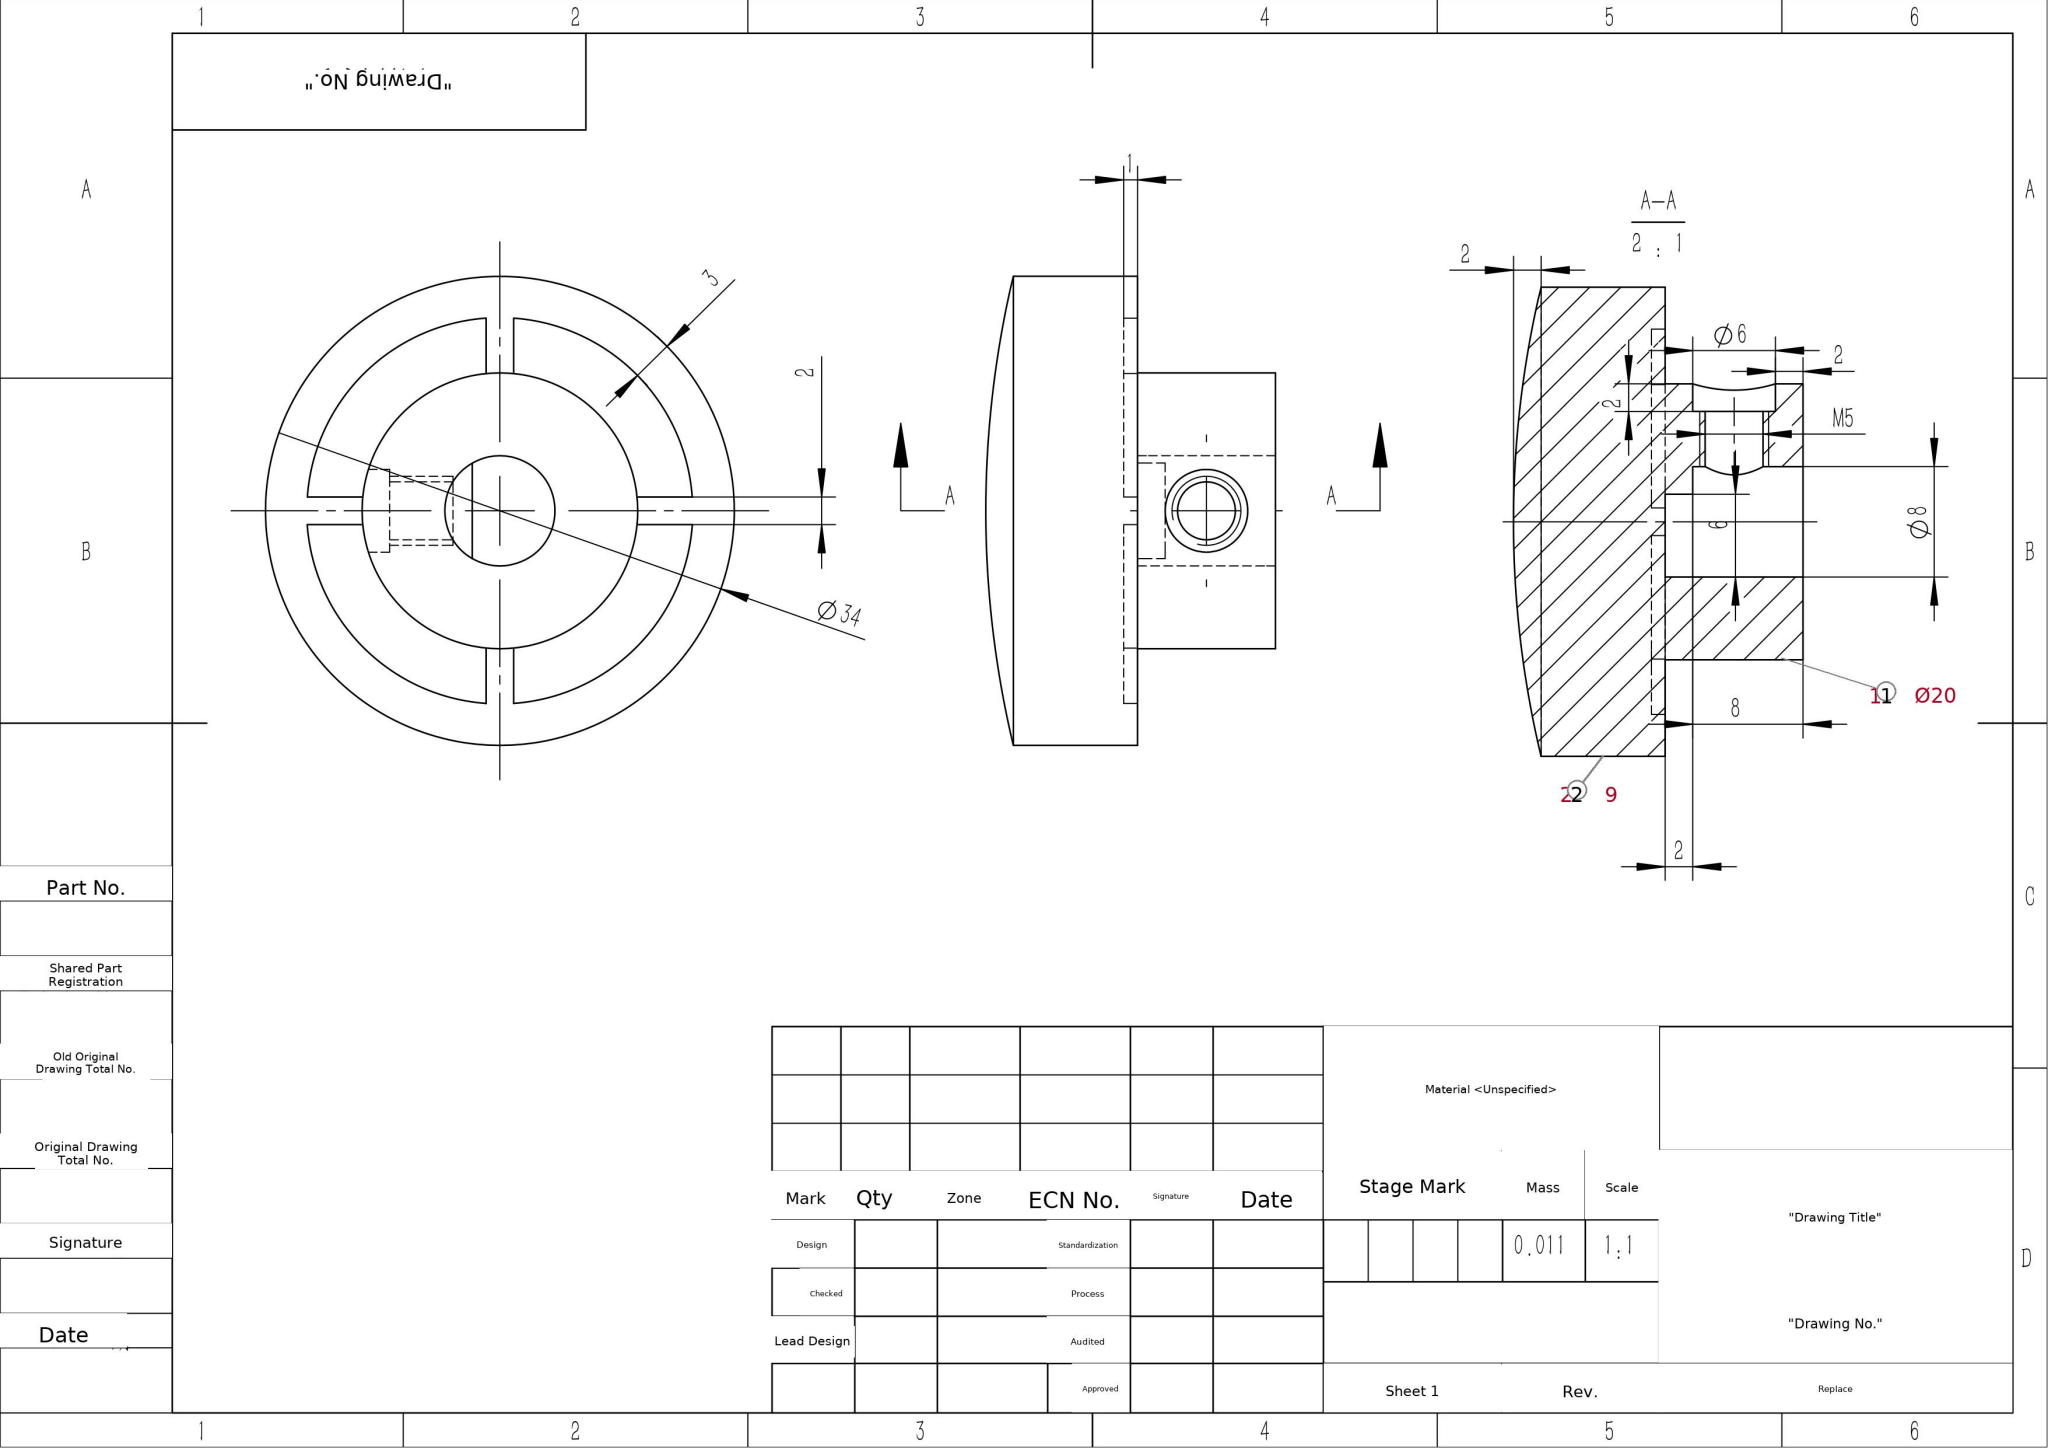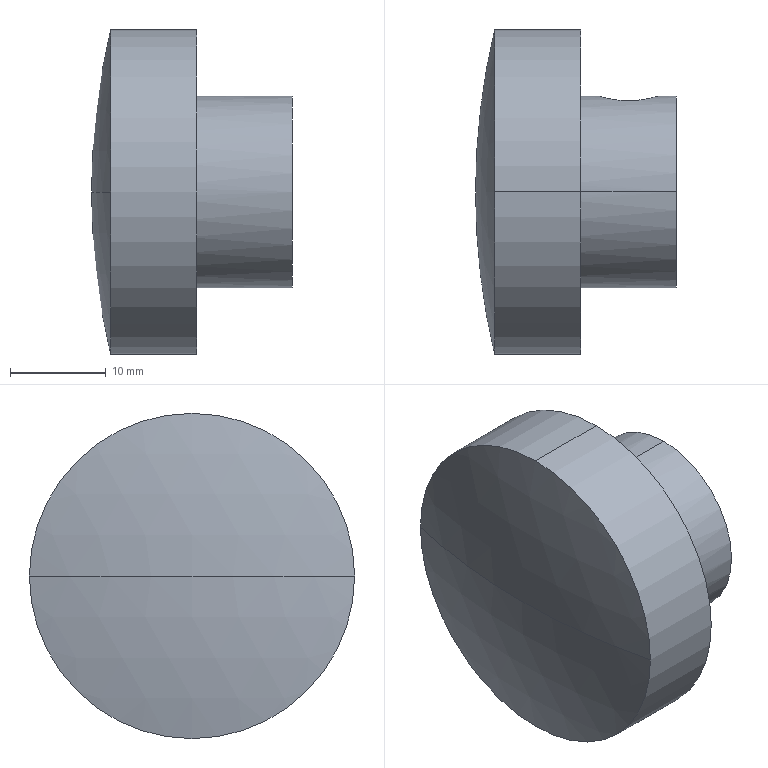Part | SolidWorks | mm | 1 solid | 34 faces | box 21 x 34 x 34 mm | volume 11362 mm3 | plane 18 | cylinder 14 | sphere 2 | commonest cylinder face diameters 28 x4 4.2 x2 6 x2 34 x2 8 x2 20 x2